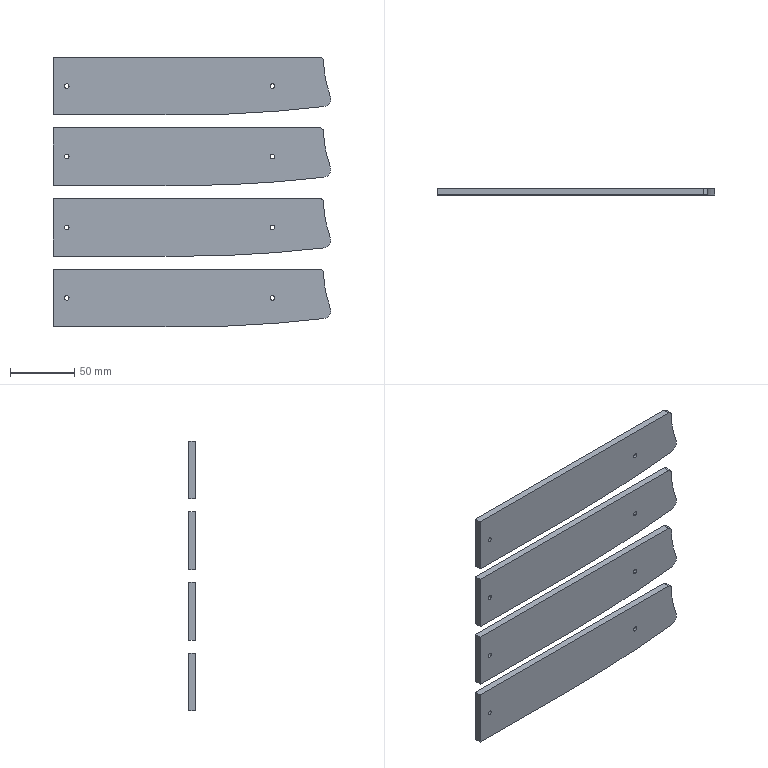CAM job | Mastercam | mm | 4 operations | part box 215.94 x 5 x 210
1. Contour (Ramp) | 3 - 3 平铣刀
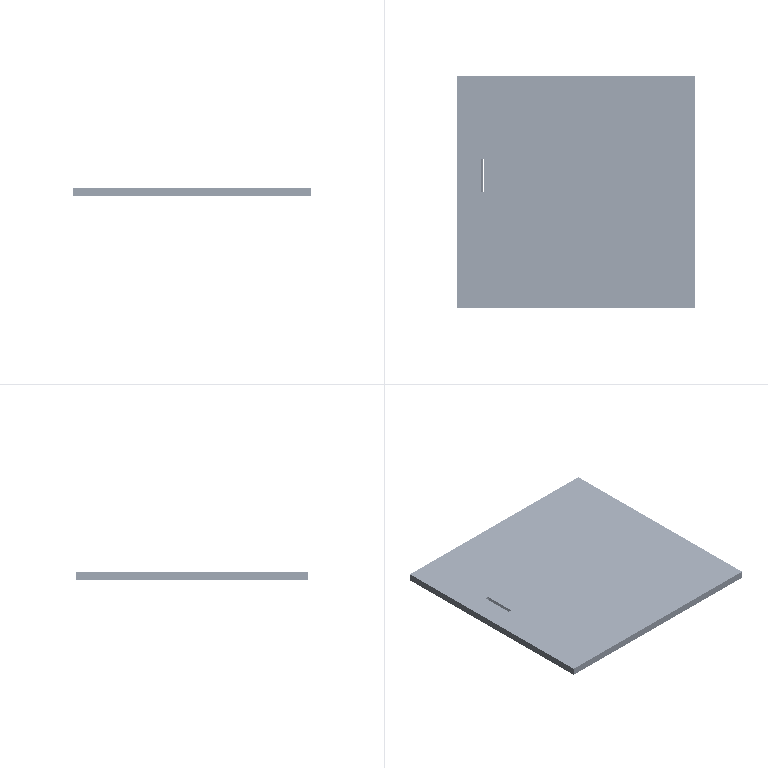2. Contour (2D) | 3 - 3 平铣刀
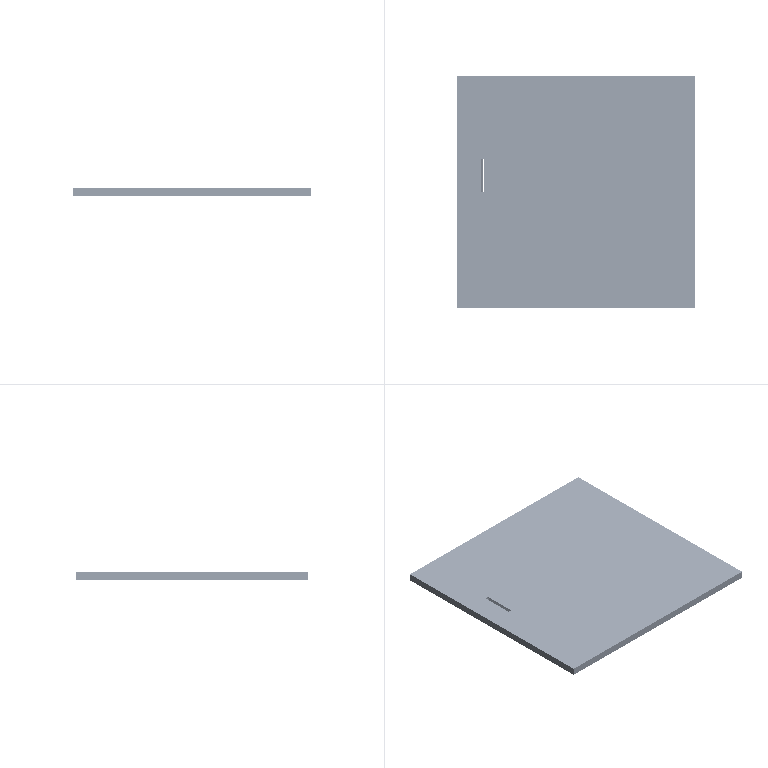3. Drill/Counterbore | 7 - 4 倒角刀
4. Contour (2D chamfer) | 7 - 4 倒角刀